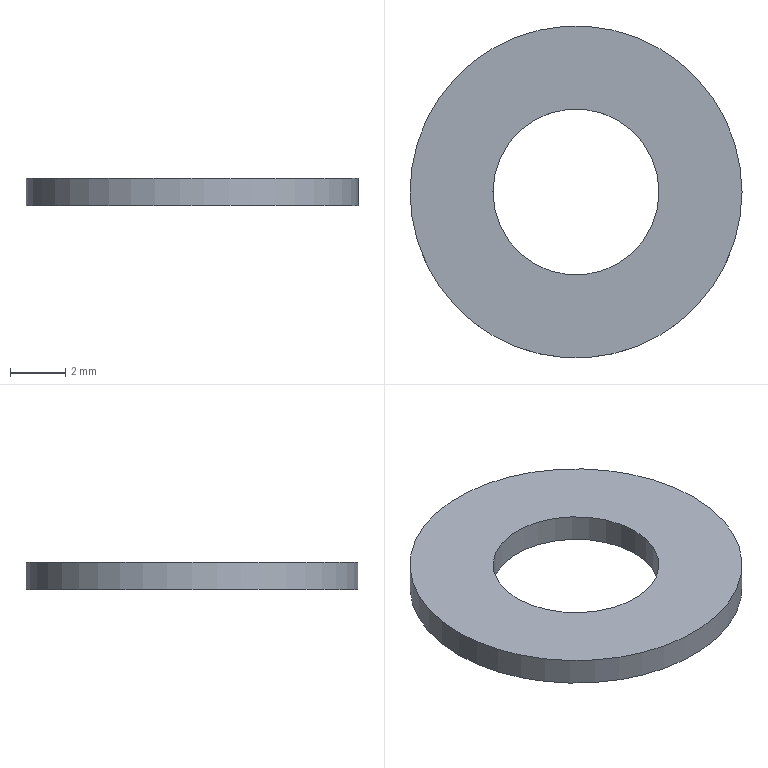Component | NX | WASHER_11 | 1 solid | 4 faces | box 12 x 12 x 1 mm | volume 85 mm3 | cylinder 2 | plane 2 | commonest cylinder face diameters 12 x1 6 x1
STEP:
#1=CARTESIAN_POINT('',(0.,0.,0.));
#2=DIRECTION('',(0.,0.,1.));
#3=DIRECTION('',(1.,0.,0.));
#4=AXIS2_PLACEMENT_3D('',#1,#2,#3);
#5=CARTESIAN_POINT('',(16.284,5.784,170.5));
#6=VERTEX_POINT('',#5);
#7=CARTESIAN_POINT('',(10.284,5.784,170.5));
#8=DIRECTION('',(0.,0.,-1.));
#9=DIRECTION('',(1.,0.,0.));
#10=AXIS2_PLACEMENT_3D('',#7,#8,#9);
#11=CIRCLE('',#10,6.);
#12=CARTESIAN_POINT('',(10.284,5.784,170.5));
#13=DIRECTION('',(0.,0.,1.));
#14=DIRECTION('',(-1.,0.,0.));
#15=AXIS2_PLACEMENT_3D('',#12,#13,#14);
#16=CYLINDRICAL_SURFACE('',#15,6.);
#17=CARTESIAN_POINT('',(9.425,0.));
#18=DIRECTION('',(-1.,0.));
#19=VECTOR('',#18,1.);
#20=LINE('',#17,#19);
#21=(GEOMETRIC_REPRESENTATION_CONTEXT(2)PARAMETRIC_REPRESENTATION_CONTEXT()REPRESENTATION_CONTEXT('',''));
#22=DEFINITIONAL_REPRESENTATION('',(#20),#21);
#23=PCURVE('',#16,#22);
#24=CARTESIAN_POINT('',(10.284,5.784,170.5));
#25=DIRECTION('',(0.,0.,-1.));
#26=DIRECTION('',(1.,0.,0.));
#27=AXIS2_PLACEMENT_3D('',#24,#25,#26);
#28=PLANE('',#27);
#29=CARTESIAN_POINT('',(0.,0.));
#30=DIRECTION('',(1.,0.));
#31=AXIS2_PLACEMENT_2D('',#29,#30);
#32=CIRCLE('',#31,6.);
#33=(GEOMETRIC_REPRESENTATION_CONTEXT(2)PARAMETRIC_REPRESENTATION_CONTEXT()REPRESENTATION_CONTEXT('',''));
#34=DEFINITIONAL_REPRESENTATION('',(#32),#33);
#35=PCURVE('',#28,#34);
#36=SURFACE_CURVE('',#11,(#23,#35),.PCURVE_S1.);
#37=EDGE_CURVE('',#6,#6,#36,.T.);
#38=ORIENTED_EDGE('',*,*,#37,.F.);
#39=CARTESIAN_POINT('',(16.284,5.784,171.5));
#40=VERTEX_POINT('',#39);
#41=CARTESIAN_POINT('',(16.284,5.784,170.5));
#42=CARTESIAN_POINT('',(16.284,5.784,171.5));
#43=B_SPLINE_CURVE_WITH_KNOTS('',1,(#41,#42),.UNSPECIFIED.,.F.,.F.,(2,2),(0.,1.),.PIECEWISE_BEZIER_KNOTS.);
#44=CARTESIAN_POINT('',(9.425,0.));
#45=DIRECTION('',(0.,1.));
#46=VECTOR('',#45,1.);
#47=LINE('',#44,#46);
#48=(GEOMETRIC_REPRESENTATION_CONTEXT(2)PARAMETRIC_REPRESENTATION_CONTEXT()REPRESENTATION_CONTEXT('',''));
#49=DEFINITIONAL_REPRESENTATION('',(#47),#48);
#50=PCURVE('',#16,#49);
#51=CARTESIAN_POINT('',(3.142,0.));
#52=DIRECTION('',(0.,1.));
#53=VECTOR('',#52,1.);
#54=LINE('',#51,#53);
#55=(GEOMETRIC_REPRESENTATION_CONTEXT(2)PARAMETRIC_REPRESENTATION_CONTEXT()REPRESENTATION_CONTEXT('',''));
#56=DEFINITIONAL_REPRESENTATION('',(#54),#55);
#57=PCURVE('',#16,#56);
#58=SEAM_CURVE('',#43,(#50,#57),.PCURVE_S1.);
#59=EDGE_CURVE('',#6,#40,#58,.T.);
#60=ORIENTED_EDGE('',*,*,#59,.T.);
#61=CARTESIAN_POINT('',(10.284,5.784,171.5));
#62=DIRECTION('',(0.,0.,-1.));
#63=DIRECTION('',(1.,0.,0.));
#64=AXIS2_PLACEMENT_3D('',#61,#62,#63);
#65=CIRCLE('',#64,6.);
#66=CARTESIAN_POINT('',(9.425,1.));
#67=DIRECTION('',(-1.,0.));
#68=VECTOR('',#67,1.);
#69=LINE('',#66,#68);
#70=(GEOMETRIC_REPRESENTATION_CONTEXT(2)PARAMETRIC_REPRESENTATION_CONTEXT()REPRESENTATION_CONTEXT('',''));
#71=DEFINITIONAL_REPRESENTATION('',(#69),#70);
#72=PCURVE('',#16,#71);
#73=CARTESIAN_POINT('',(10.284,5.784,171.5));
#74=DIRECTION('',(0.,0.,-1.));
#75=DIRECTION('',(1.,0.,0.));
#76=AXIS2_PLACEMENT_3D('',#73,#74,#75);
#77=PLANE('',#76);
#78=CARTESIAN_POINT('',(0.,0.));
#79=DIRECTION('',(1.,0.));
#80=AXIS2_PLACEMENT_2D('',#78,#79);
#81=CIRCLE('',#80,6.);
#82=(GEOMETRIC_REPRESENTATION_CONTEXT(2)PARAMETRIC_REPRESENTATION_CONTEXT()REPRESENTATION_CONTEXT('',''));
#83=DEFINITIONAL_REPRESENTATION('',(#81),#82);
#84=PCURVE('',#77,#83);
#85=SURFACE_CURVE('',#65,(#72,#84),.PCURVE_S1.);
#86=EDGE_CURVE('',#40,#40,#85,.T.);
#87=ORIENTED_EDGE('',*,*,#86,.T.);
#88=ORIENTED_EDGE('',*,*,#59,.F.);
#89=EDGE_LOOP('',(#38,#60,#87,#88));
#90=FACE_BOUND('',#89,.T.);
#91=ADVANCED_FACE('',(#90),#16,.T.);
#92=CARTESIAN_POINT('',(13.284,5.784,170.5));
#93=VERTEX_POINT('',#92);
#94=CARTESIAN_POINT('',(10.284,5.784,170.5));
#95=DIRECTION('',(0.,0.,-1.));
#96=DIRECTION('',(1.,0.,0.));
#97=AXIS2_PLACEMENT_3D('',#94,#95,#96);
#98=CIRCLE('',#97,3.);
#99=CARTESIAN_POINT('',(10.284,5.784,170.5));
#100=DIRECTION('',(0.,0.,1.));
#101=DIRECTION('',(-1.,0.,0.));
#102=AXIS2_PLACEMENT_3D('',#99,#100,#101);
#103=CYLINDRICAL_SURFACE('',#102,3.);
#104=CARTESIAN_POINT('',(9.425,0.));
#105=DIRECTION('',(-1.,0.));
#106=VECTOR('',#105,1.);
#107=LINE('',#104,#106);
#108=(GEOMETRIC_REPRESENTATION_CONTEXT(2)PARAMETRIC_REPRESENTATION_CONTEXT()REPRESENTATION_CONTEXT('',''));
#109=DEFINITIONAL_REPRESENTATION('',(#107),#108);
#110=PCURVE('',#103,#109);
#111=CARTESIAN_POINT('',(0.,0.));
#112=DIRECTION('',(1.,0.));
#113=AXIS2_PLACEMENT_2D('',#111,#112);
#114=CIRCLE('',#113,3.);
#115=(GEOMETRIC_REPRESENTATION_CONTEXT(2)PARAMETRIC_REPRESENTATION_CONTEXT()REPRESENTATION_CONTEXT('',''));
#116=DEFINITIONAL_REPRESENTATION('',(#114),#115);
#117=PCURVE('',#28,#116);
#118=SURFACE_CURVE('',#98,(#110,#117),.PCURVE_S1.);
#119=EDGE_CURVE('',#93,#93,#118,.T.);
#120=ORIENTED_EDGE('',*,*,#119,.F.);
#121=CARTESIAN_POINT('',(13.284,5.784,171.5));
#122=VERTEX_POINT('',#121);
#123=CARTESIAN_POINT('',(13.284,5.784,170.5));
#124=CARTESIAN_POINT('',(13.284,5.784,171.5));
#125=B_SPLINE_CURVE_WITH_KNOTS('',1,(#123,#124),.UNSPECIFIED.,.F.,.F.,(2,2),(0.,1.),.PIECEWISE_BEZIER_KNOTS.);
#126=CARTESIAN_POINT('',(9.425,0.));
#127=DIRECTION('',(0.,1.));
#128=VECTOR('',#127,1.);
#129=LINE('',#126,#128);
#130=(GEOMETRIC_REPRESENTATION_CONTEXT(2)PARAMETRIC_REPRESENTATION_CONTEXT()REPRESENTATION_CONTEXT('',''));
#131=DEFINITIONAL_REPRESENTATION('',(#129),#130);
#132=PCURVE('',#103,#131);
#133=CARTESIAN_POINT('',(3.142,0.));
#134=DIRECTION('',(0.,1.));
#135=VECTOR('',#134,1.);
#136=LINE('',#133,#135);
#137=(GEOMETRIC_REPRESENTATION_CONTEXT(2)PARAMETRIC_REPRESENTATION_CONTEXT()REPRESENTATION_CONTEXT('',''));
#138=DEFINITIONAL_REPRESENTATION('',(#136),#137);
#139=PCURVE('',#103,#138);
#140=SEAM_CURVE('',#125,(#132,#139),.PCURVE_S1.);
#141=EDGE_CURVE('',#93,#122,#140,.T.);
#142=ORIENTED_EDGE('',*,*,#141,.T.);
#143=CARTESIAN_POINT('',(10.284,5.784,171.5));
#144=DIRECTION('',(0.,0.,-1.));
#145=DIRECTION('',(1.,0.,0.));
#146=AXIS2_PLACEMENT_3D('',#143,#144,#145);
#147=CIRCLE('',#146,3.);
#148=CARTESIAN_POINT('',(9.425,1.));
#149=DIRECTION('',(-1.,0.));
#150=VECTOR('',#149,1.);
#151=LINE('',#148,#150);
#152=(GEOMETRIC_REPRESENTATION_CONTEXT(2)PARAMETRIC_REPRESENTATION_CONTEXT()REPRESENTATION_CONTEXT('',''));
#153=DEFINITIONAL_REPRESENTATION('',(#151),#152);
#154=PCURVE('',#103,#153);
#155=CARTESIAN_POINT('',(0.,0.));
#156=DIRECTION('',(1.,0.));
#157=AXIS2_PLACEMENT_2D('',#155,#156);
#158=CIRCLE('',#157,3.);
#159=(GEOMETRIC_REPRESENTATION_CONTEXT(2)PARAMETRIC_REPRESENTATION_CONTEXT()REPRESENTATION_CONTEXT('',''));
#160=DEFINITIONAL_REPRESENTATION('',(#158),#159);
#161=PCURVE('',#77,#160);
#162=SURFACE_CURVE('',#147,(#154,#161),.PCURVE_S1.);
#163=EDGE_CURVE('',#122,#122,#162,.T.);
#164=ORIENTED_EDGE('',*,*,#163,.T.);
#165=ORIENTED_EDGE('',*,*,#141,.F.);
#166=EDGE_LOOP('',(#120,#142,#164,#165));
#167=FACE_BOUND('',#166,.F.);
#168=ADVANCED_FACE('',(#167),#103,.F.);
#169=ORIENTED_EDGE('',*,*,#37,.T.);
#170=EDGE_LOOP('',(#169));
#171=FACE_BOUND('',#170,.T.);
#172=ORIENTED_EDGE('',*,*,#119,.F.);
#173=EDGE_LOOP('',(#172));
#174=FACE_BOUND('',#173,.T.);
#175=ADVANCED_FACE('',(#171,#174),#28,.T.);
#176=ORIENTED_EDGE('',*,*,#86,.F.);
#177=EDGE_LOOP('',(#176));
#178=FACE_BOUND('',#177,.T.);
#179=ORIENTED_EDGE('',*,*,#163,.T.);
#180=EDGE_LOOP('',(#179));
#181=FACE_BOUND('',#180,.T.);
#182=ADVANCED_FACE('',(#178,#181),#77,.F.);
#183=CLOSED_SHELL('',(#91,#168,#175,#182));
#184=MANIFOLD_SOLID_BREP('',#183);
#185=(LENGTH_UNIT()NAMED_UNIT(*)SI_UNIT(.MILLI.,.METRE.));
#186=UNCERTAINTY_MEASURE_WITH_UNIT(LENGTH_MEASURE(0.00001),#185,'','');
#187=(NAMED_UNIT(*)PLANE_ANGLE_UNIT()SI_UNIT($,.RADIAN.));
#188=(NAMED_UNIT(*)SI_UNIT($,.STERADIAN.)SOLID_ANGLE_UNIT());
#189=(GEOMETRIC_REPRESENTATION_CONTEXT(3)GLOBAL_UNCERTAINTY_ASSIGNED_CONTEXT((#186))GLOBAL_UNIT_ASSIGNED_CONTEXT((#185,#187,#188))REPRESENTATION_CONTEXT('',''));
#190=ADVANCED_BREP_SHAPE_REPRESENTATION('',(#4,#184),#189);